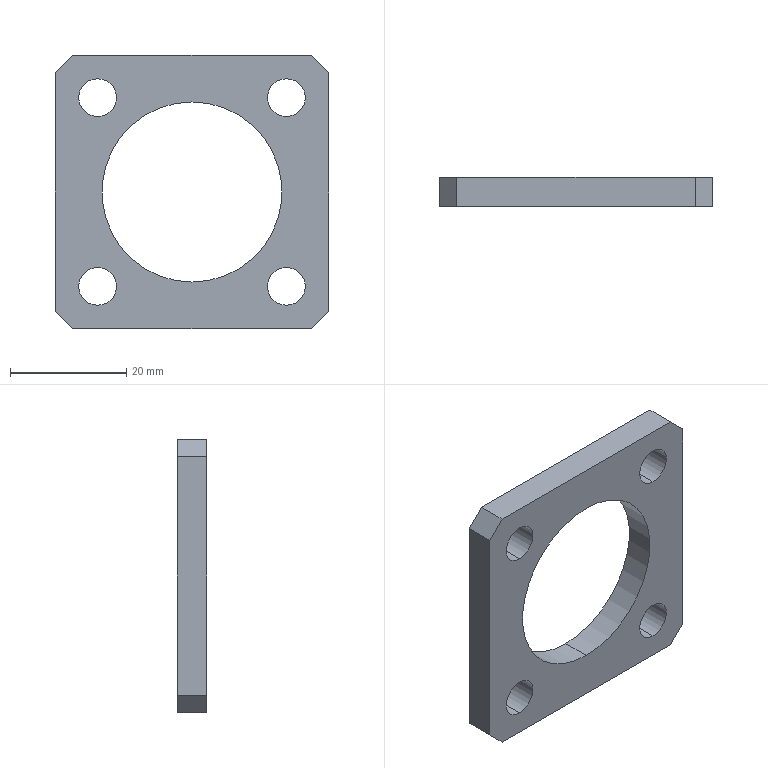Component | SolidWorks | F12529-M5116-1 | 1 solid | 20 faces | box 47 x 5 x 47 mm | volume 6518 mm3 | cylinder 10 | plane 10 | commonest cylinder face diameters 6.5 x8 31 x2
build123d program:
from build123d import *

# Parameters (mm, degrees)
SKETCH1_W           = 47
SKETCH1_H           = 47
BOSS_EXTRUDE1_DEPTH = 5
CHAMFER1_SIZE       = 3
SKETCH2_R           = 15.5
CUT_EXTRUDE1_DEPTH  = 5
SKETCH3_R           = 3.25
CUT_EXTRUDE2_DEPTH  = 5


with BuildPart() as part:
    # Sketch1 → Boss-Extrude1 (new body)
    with BuildSketch(Plane(origin=(0, 0, 0), x_dir=(1, 0, 0), z_dir=(0, 1, 0))):
        Rectangle(SKETCH1_W, SKETCH1_H)
    extrude(amount=BOSS_EXTRUDE1_DEPTH)

    # Chamfer1
    chamfer1_edges = [part.edges().sort_by_distance(p)[0] for p in [
        (-23.5, 2.5, -23.5),
        (23.5, 2.5, -23.5),
        (23.5, 2.5, 23.5),
        (-23.5, 2.5, 23.5),
    ]]
    chamfer(chamfer1_edges, length=CHAMFER1_SIZE)

    # Sketch2 → Cut-Extrude1 (cut)
    with BuildSketch(Plane(origin=(0, 5, 0), x_dir=(1, 0, 0), z_dir=(0, 1, 0))):
        with Locations(Location((0, 0, 0), (0, 0, 270))):
            Circle(SKETCH2_R)
    extrude(amount=-CUT_EXTRUDE1_DEPTH, mode=Mode.SUBTRACT)

    # Sketch3 → Cut-Extrude2 (cut)
    with BuildSketch(Plane(origin=(0, 5, 0), x_dir=(1, 0, 0), z_dir=(0, 1, 0))):
        with Locations(Location((16.25, 16.25, 0), (0, 0, 270))):
            Circle(SKETCH3_R)
        with Locations(Location((16.25, -16.25, 0), (0, 0, 270))):
            Circle(SKETCH3_R)
    cut_extrude2 = extrude(amount=-CUT_EXTRUDE2_DEPTH, mode=Mode.SUBTRACT)

    # Mirror1: Cut-Extrude2 across plane
    add(cut_extrude2.mirror(Plane(origin=(0, 0, 0), x_dir=(0, 0, 1), z_dir=(1, 0, 0))), mode=Mode.SUBTRACT)


solid = part.part

# Placed as in the assembly
solid = solid.moved(Location((0, -5, 0), (0, 0, 0)))
STEP:
#1=COLOUR_RGB('',0.7922,0.8196,0.9333);
#2=FILL_AREA_STYLE_COLOUR('',#1);
#3=FILL_AREA_STYLE('',(#2));
#4=SURFACE_STYLE_FILL_AREA(#3);
#5=SURFACE_SIDE_STYLE('',(#4));
#6=SURFACE_STYLE_USAGE(.BOTH.,#5);
#7=PRESENTATION_STYLE_ASSIGNMENT((#6));
#8=CARTESIAN_POINT('',(-0.6398,-0.1969,0.7677));
#9=VERTEX_POINT('',#8);
#10=CARTESIAN_POINT('',(-0.6398,-0.1969,0.5118));
#11=VERTEX_POINT('',#10);
#12=CARTESIAN_POINT('',(-0.6398,-0.1969,0.6398));
#13=DIRECTION('',(0.,-1.,0.));
#14=DIRECTION('',(0.,0.,1.));
#15=AXIS2_PLACEMENT_3D('',#12,#13,#14);
#16=CIRCLE('',#15,0.128);
#17=EDGE_CURVE('',#9,#11,#16,.T.);
#18=ORIENTED_EDGE('',*,*,#17,.T.);
#19=CARTESIAN_POINT('',(-0.6398,0.,0.5118));
#20=VERTEX_POINT('',#19);
#21=CARTESIAN_POINT('',(-0.6398,-0.1969,0.5118));
#22=DIRECTION('',(0.,1.,0.));
#23=VECTOR('',#22,39.37);
#24=LINE('',#21,#23);
#25=EDGE_CURVE('',#11,#20,#24,.T.);
#26=ORIENTED_EDGE('',*,*,#25,.T.);
#27=CARTESIAN_POINT('',(-0.6398,0.,0.7677));
#28=VERTEX_POINT('',#27);
#29=CARTESIAN_POINT('',(-0.6398,0.,0.6398));
#30=DIRECTION('',(0.,-1.,0.));
#31=DIRECTION('',(0.,0.,1.));
#32=AXIS2_PLACEMENT_3D('',#29,#30,#31);
#33=CIRCLE('',#32,0.128);
#34=EDGE_CURVE('',#28,#20,#33,.T.);
#35=ORIENTED_EDGE('',*,*,#34,.F.);
#36=CARTESIAN_POINT('',(-0.6398,-0.1969,0.7677));
#37=DIRECTION('',(0.,1.,0.));
#38=VECTOR('',#37,39.37);
#39=LINE('',#36,#38);
#40=EDGE_CURVE('',#9,#28,#39,.T.);
#41=ORIENTED_EDGE('',*,*,#40,.F.);
#42=EDGE_LOOP('',(#18,#26,#35,#41));
#43=FACE_OUTER_BOUND('',#42,.T.);
#44=CARTESIAN_POINT('',(-0.6398,-0.1969,0.6398));
#45=DIRECTION('',(0.,1.,0.));
#46=DIRECTION('',(0.,0.,1.));
#47=AXIS2_PLACEMENT_3D('',#44,#45,#46);
#48=CYLINDRICAL_SURFACE('',#47,0.128);
#49=ADVANCED_FACE('',(#43),#48,.F.);
#50=CARTESIAN_POINT('',(-0.6398,-0.1969,-0.5118));
#51=VERTEX_POINT('',#50);
#52=CARTESIAN_POINT('',(-0.6398,-0.1969,-0.7677));
#53=VERTEX_POINT('',#52);
#54=CARTESIAN_POINT('',(-0.6398,-0.1969,-0.6398));
#55=DIRECTION('',(0.,-1.,0.));
#56=DIRECTION('',(0.,0.,1.));
#57=AXIS2_PLACEMENT_3D('',#54,#55,#56);
#58=CIRCLE('',#57,0.128);
#59=EDGE_CURVE('',#51,#53,#58,.T.);
#60=ORIENTED_EDGE('',*,*,#59,.T.);
#61=CARTESIAN_POINT('',(-0.6398,0.,-0.7677));
#62=VERTEX_POINT('',#61);
#63=CARTESIAN_POINT('',(-0.6398,-0.1969,-0.7677));
#64=DIRECTION('',(0.,1.,0.));
#65=VECTOR('',#64,39.37);
#66=LINE('',#63,#65);
#67=EDGE_CURVE('',#53,#62,#66,.T.);
#68=ORIENTED_EDGE('',*,*,#67,.T.);
#69=CARTESIAN_POINT('',(-0.6398,0.,-0.5118));
#70=VERTEX_POINT('',#69);
#71=CARTESIAN_POINT('',(-0.6398,0.,-0.6398));
#72=DIRECTION('',(0.,-1.,0.));
#73=DIRECTION('',(0.,0.,1.));
#74=AXIS2_PLACEMENT_3D('',#71,#72,#73);
#75=CIRCLE('',#74,0.128);
#76=EDGE_CURVE('',#70,#62,#75,.T.);
#77=ORIENTED_EDGE('',*,*,#76,.F.);
#78=CARTESIAN_POINT('',(-0.6398,-0.1969,-0.5118));
#79=DIRECTION('',(0.,1.,0.));
#80=VECTOR('',#79,39.37);
#81=LINE('',#78,#80);
#82=EDGE_CURVE('',#51,#70,#81,.T.);
#83=ORIENTED_EDGE('',*,*,#82,.F.);
#84=EDGE_LOOP('',(#60,#68,#77,#83));
#85=FACE_OUTER_BOUND('',#84,.T.);
#86=CARTESIAN_POINT('',(-0.6398,-0.1969,-0.6398));
#87=DIRECTION('',(0.,1.,0.));
#88=DIRECTION('',(0.,0.,1.));
#89=AXIS2_PLACEMENT_3D('',#86,#87,#88);
#90=CYLINDRICAL_SURFACE('',#89,0.128);
#91=ADVANCED_FACE('',(#85),#90,.F.);
#92=CARTESIAN_POINT('',(0.6398,-0.1969,0.5118));
#93=VERTEX_POINT('',#92);
#94=CARTESIAN_POINT('',(0.6398,-0.1969,0.7677));
#95=VERTEX_POINT('',#94);
#96=CARTESIAN_POINT('',(0.6398,-0.1969,0.6398));
#97=DIRECTION('',(0.,1.,0.));
#98=DIRECTION('',(0.,0.,1.));
#99=AXIS2_PLACEMENT_3D('',#96,#97,#98);
#100=CIRCLE('',#99,0.128);
#101=EDGE_CURVE('',#93,#95,#100,.T.);
#102=ORIENTED_EDGE('',*,*,#101,.F.);
#103=CARTESIAN_POINT('',(0.6398,0.,0.5118));
#104=VERTEX_POINT('',#103);
#105=CARTESIAN_POINT('',(0.6398,-0.1969,0.5118));
#106=DIRECTION('',(0.,1.,0.));
#107=VECTOR('',#106,39.37);
#108=LINE('',#105,#107);
#109=EDGE_CURVE('',#93,#104,#108,.T.);
#110=ORIENTED_EDGE('',*,*,#109,.T.);
#111=CARTESIAN_POINT('',(0.6398,0.,0.7677));
#112=VERTEX_POINT('',#111);
#113=CARTESIAN_POINT('',(0.6398,0.,0.6398));
#114=DIRECTION('',(0.,1.,0.));
#115=DIRECTION('',(0.,0.,1.));
#116=AXIS2_PLACEMENT_3D('',#113,#114,#115);
#117=CIRCLE('',#116,0.128);
#118=EDGE_CURVE('',#104,#112,#117,.T.);
#119=ORIENTED_EDGE('',*,*,#118,.T.);
#120=CARTESIAN_POINT('',(0.6398,-0.1969,0.7677));
#121=DIRECTION('',(0.,1.,0.));
#122=VECTOR('',#121,39.37);
#123=LINE('',#120,#122);
#124=EDGE_CURVE('',#95,#112,#123,.T.);
#125=ORIENTED_EDGE('',*,*,#124,.F.);
#126=EDGE_LOOP('',(#102,#110,#119,#125));
#127=FACE_OUTER_BOUND('',#126,.T.);
#128=CARTESIAN_POINT('',(0.6398,-0.1969,0.6398));
#129=DIRECTION('',(0.,1.,0.));
#130=DIRECTION('',(0.,0.,1.));
#131=AXIS2_PLACEMENT_3D('',#128,#129,#130);
#132=CYLINDRICAL_SURFACE('',#131,0.128);
#133=ADVANCED_FACE('',(#127),#132,.F.);
#134=CARTESIAN_POINT('',(0.6398,-0.1969,-0.7677));
#135=VERTEX_POINT('',#134);
#136=CARTESIAN_POINT('',(0.6398,-0.1969,-0.5118));
#137=VERTEX_POINT('',#136);
#138=CARTESIAN_POINT('',(0.6398,-0.1969,-0.6398));
#139=DIRECTION('',(0.,1.,0.));
#140=DIRECTION('',(0.,0.,1.));
#141=AXIS2_PLACEMENT_3D('',#138,#139,#140);
#142=CIRCLE('',#141,0.128);
#143=EDGE_CURVE('',#135,#137,#142,.T.);
#144=ORIENTED_EDGE('',*,*,#143,.F.);
#145=CARTESIAN_POINT('',(0.6398,0.,-0.7677));
#146=VERTEX_POINT('',#145);
#147=CARTESIAN_POINT('',(0.6398,-0.1969,-0.7677));
#148=DIRECTION('',(0.,1.,0.));
#149=VECTOR('',#148,39.37);
#150=LINE('',#147,#149);
#151=EDGE_CURVE('',#135,#146,#150,.T.);
#152=ORIENTED_EDGE('',*,*,#151,.T.);
#153=CARTESIAN_POINT('',(0.6398,0.,-0.5118));
#154=VERTEX_POINT('',#153);
#155=CARTESIAN_POINT('',(0.6398,0.,-0.6398));
#156=DIRECTION('',(0.,1.,0.));
#157=DIRECTION('',(0.,0.,1.));
#158=AXIS2_PLACEMENT_3D('',#155,#156,#157);
#159=CIRCLE('',#158,0.128);
#160=EDGE_CURVE('',#146,#154,#159,.T.);
#161=ORIENTED_EDGE('',*,*,#160,.T.);
#162=CARTESIAN_POINT('',(0.6398,-0.1969,-0.5118));
#163=DIRECTION('',(0.,1.,0.));
#164=VECTOR('',#163,39.37);
#165=LINE('',#162,#164);
#166=EDGE_CURVE('',#137,#154,#165,.T.);
#167=ORIENTED_EDGE('',*,*,#166,.F.);
#168=EDGE_LOOP('',(#144,#152,#161,#167));
#169=FACE_OUTER_BOUND('',#168,.T.);
#170=CARTESIAN_POINT('',(0.6398,-0.1969,-0.6398));
#171=DIRECTION('',(0.,1.,0.));
#172=DIRECTION('',(0.,0.,1.));
#173=AXIS2_PLACEMENT_3D('',#170,#171,#172);
#174=CYLINDRICAL_SURFACE('',#173,0.128);
#175=ADVANCED_FACE('',(#169),#174,.F.);
#176=CARTESIAN_POINT('',(0.,-0.1969,-0.6102));
#177=VERTEX_POINT('',#176);
#178=CARTESIAN_POINT('',(-0.,-0.1969,0.6102));
#179=VERTEX_POINT('',#178);
#180=CARTESIAN_POINT('',(-0.,-0.1969,-0.));
#181=DIRECTION('',(0.,1.,0.));
#182=DIRECTION('',(0.,0.,1.));
#183=AXIS2_PLACEMENT_3D('',#180,#181,#182);
#184=CIRCLE('',#183,0.6102);
#185=EDGE_CURVE('',#177,#179,#184,.T.);
#186=ORIENTED_EDGE('',*,*,#185,.F.);
#187=CARTESIAN_POINT('',(0.,0.,-0.6102));
#188=VERTEX_POINT('',#187);
#189=CARTESIAN_POINT('',(0.,-0.1969,-0.6102));
#190=DIRECTION('',(0.,1.,0.));
#191=VECTOR('',#190,39.37);
#192=LINE('',#189,#191);
#193=EDGE_CURVE('',#177,#188,#192,.T.);
#194=ORIENTED_EDGE('',*,*,#193,.T.);
#195=CARTESIAN_POINT('',(-0.,0.,0.6102));
#196=VERTEX_POINT('',#195);
#197=CARTESIAN_POINT('',(-0.,0.,-0.));
#198=DIRECTION('',(0.,1.,0.));
#199=DIRECTION('',(0.,0.,1.));
#200=AXIS2_PLACEMENT_3D('',#197,#198,#199);
#201=CIRCLE('',#200,0.6102);
#202=EDGE_CURVE('',#188,#196,#201,.T.);
#203=ORIENTED_EDGE('',*,*,#202,.T.);
#204=CARTESIAN_POINT('',(-0.,-0.1969,0.6102));
#205=DIRECTION('',(0.,1.,0.));
#206=VECTOR('',#205,39.37);
#207=LINE('',#204,#206);
#208=EDGE_CURVE('',#179,#196,#207,.T.);
#209=ORIENTED_EDGE('',*,*,#208,.F.);
#210=EDGE_LOOP('',(#186,#194,#203,#209));
#211=FACE_OUTER_BOUND('',#210,.T.);
#212=CARTESIAN_POINT('',(-0.,-0.1969,-0.));
#213=DIRECTION('',(0.,1.,0.));
#214=DIRECTION('',(0.,0.,1.));
#215=AXIS2_PLACEMENT_3D('',#212,#213,#214);
#216=CYLINDRICAL_SURFACE('',#215,0.6102);
#217=ADVANCED_FACE('',(#211),#216,.F.);
#218=ORIENTED_EDGE('',*,*,#76,.T.);
#219=CARTESIAN_POINT('',(-0.6398,0.,-0.6398));
#220=DIRECTION('',(0.,-1.,0.));
#221=DIRECTION('',(0.,0.,1.));
#222=AXIS2_PLACEMENT_3D('',#219,#220,#221);
#223=CIRCLE('',#222,0.128);
#224=EDGE_CURVE('',#62,#70,#223,.T.);
#225=ORIENTED_EDGE('',*,*,#224,.T.);
#226=EDGE_LOOP('',(#218,#225));
#227=FACE_BOUND('',#226,.T.);
#228=CARTESIAN_POINT('',(0.6398,0.,0.6398));
#229=DIRECTION('',(0.,1.,0.));
#230=DIRECTION('',(0.,0.,1.));
#231=AXIS2_PLACEMENT_3D('',#228,#229,#230);
#232=CIRCLE('',#231,0.128);
#233=EDGE_CURVE('',#112,#104,#232,.T.);
#234=ORIENTED_EDGE('',*,*,#233,.F.);
#235=ORIENTED_EDGE('',*,*,#118,.F.);
#236=EDGE_LOOP('',(#234,#235));
#237=FACE_BOUND('',#236,.T.);
#238=CARTESIAN_POINT('',(0.6398,0.,-0.6398));
#239=DIRECTION('',(0.,1.,0.));
#240=DIRECTION('',(0.,0.,1.));
#241=AXIS2_PLACEMENT_3D('',#238,#239,#240);
#242=CIRCLE('',#241,0.128);
#243=EDGE_CURVE('',#154,#146,#242,.T.);
#244=ORIENTED_EDGE('',*,*,#243,.F.);
#245=ORIENTED_EDGE('',*,*,#160,.F.);
#246=EDGE_LOOP('',(#244,#245));
#247=FACE_BOUND('',#246,.T.);
#248=CARTESIAN_POINT('',(-0.,0.,-0.));
#249=DIRECTION('',(0.,1.,0.));
#250=DIRECTION('',(0.,0.,1.));
#251=AXIS2_PLACEMENT_3D('',#248,#249,#250);
#252=CIRCLE('',#251,0.6102);
#253=EDGE_CURVE('',#196,#188,#252,.T.);
#254=ORIENTED_EDGE('',*,*,#253,.F.);
#255=ORIENTED_EDGE('',*,*,#202,.F.);
#256=EDGE_LOOP('',(#254,#255));
#257=FACE_BOUND('',#256,.T.);
#258=CARTESIAN_POINT('',(-0.9252,0.,-0.8071));
#259=VERTEX_POINT('',#258);
#260=CARTESIAN_POINT('',(-0.9252,0.,0.8071));
#261=VERTEX_POINT('',#260);
#262=CARTESIAN_POINT('',(-0.9252,0.,-0.9252));
#263=DIRECTION('',(0.,0.,1.));
#264=VECTOR('',#263,39.37);
#265=LINE('',#262,#264);
#266=EDGE_CURVE('',#259,#261,#265,.T.);
#267=ORIENTED_EDGE('',*,*,#266,.T.);
#268=CARTESIAN_POINT('',(-0.8071,0.,0.9252));
#269=VERTEX_POINT('',#268);
#270=CARTESIAN_POINT('',(-0.8661,0.,0.8661));
#271=DIRECTION('',(0.7071,0.,0.7071));
#272=VECTOR('',#271,39.37);
#273=LINE('',#270,#272);
#274=EDGE_CURVE('',#261,#269,#273,.T.);
#275=ORIENTED_EDGE('',*,*,#274,.T.);
#276=CARTESIAN_POINT('',(0.8071,0.,0.9252));
#277=VERTEX_POINT('',#276);
#278=CARTESIAN_POINT('',(-0.9252,0.,0.9252));
#279=DIRECTION('',(1.,0.,0.));
#280=VECTOR('',#279,39.37);
#281=LINE('',#278,#280);
#282=EDGE_CURVE('',#269,#277,#281,.T.);
#283=ORIENTED_EDGE('',*,*,#282,.T.);
#284=CARTESIAN_POINT('',(0.9252,0.,0.8071));
#285=VERTEX_POINT('',#284);
#286=CARTESIAN_POINT('',(-0.05906,0.,1.791));
#287=DIRECTION('',(0.7071,0.,-0.7071));
#288=VECTOR('',#287,39.37);
#289=LINE('',#286,#288);
#290=EDGE_CURVE('',#277,#285,#289,.T.);
#291=ORIENTED_EDGE('',*,*,#290,.T.);
#292=CARTESIAN_POINT('',(0.9252,0.,-0.8071));
#293=VERTEX_POINT('',#292);
#294=CARTESIAN_POINT('',(0.9252,0.,-0.9252));
#295=DIRECTION('',(-0.,0.,-1.));
#296=VECTOR('',#295,39.37);
#297=LINE('',#294,#296);
#298=EDGE_CURVE('',#285,#293,#297,.T.);
#299=ORIENTED_EDGE('',*,*,#298,.T.);
#300=CARTESIAN_POINT('',(0.8071,0.,-0.9252));
#301=VERTEX_POINT('',#300);
#302=CARTESIAN_POINT('',(0.8661,0.,-0.8661));
#303=DIRECTION('',(-0.7071,0.,-0.7071));
#304=VECTOR('',#303,39.37);
#305=LINE('',#302,#304);
#306=EDGE_CURVE('',#293,#301,#305,.T.);
#307=ORIENTED_EDGE('',*,*,#306,.T.);
#308=CARTESIAN_POINT('',(-0.8071,0.,-0.9252));
#309=VERTEX_POINT('',#308);
#310=CARTESIAN_POINT('',(-0.9252,0.,-0.9252));
#311=DIRECTION('',(-1.,0.,0.));
#312=VECTOR('',#311,39.37);
#313=LINE('',#310,#312);
#314=EDGE_CURVE('',#301,#309,#313,.T.);
#315=ORIENTED_EDGE('',*,*,#314,.T.);
#316=CARTESIAN_POINT('',(-1.791,0.,0.05906));
#317=DIRECTION('',(-0.7071,0.,0.7071));
#318=VECTOR('',#317,39.37);
#319=LINE('',#316,#318);
#320=EDGE_CURVE('',#309,#259,#319,.T.);
#321=ORIENTED_EDGE('',*,*,#320,.T.);
#322=EDGE_LOOP('',(#267,#275,#283,#291,#299,#307,#315,#321));
#323=FACE_OUTER_BOUND('',#322,.T.);
#324=ORIENTED_EDGE('',*,*,#34,.T.);
#325=CARTESIAN_POINT('',(-0.6398,0.,0.6398));
#326=DIRECTION('',(0.,-1.,0.));
#327=DIRECTION('',(0.,0.,1.));
#328=AXIS2_PLACEMENT_3D('',#325,#326,#327);
#329=CIRCLE('',#328,0.128);
#330=EDGE_CURVE('',#20,#28,#329,.T.);
#331=ORIENTED_EDGE('',*,*,#330,.T.);
#332=EDGE_LOOP('',(#324,#331));
#333=FACE_BOUND('',#332,.T.);
#334=CARTESIAN_POINT('',(-0.9252,0.,0.9252));
#335=DIRECTION('',(0.,1.,0.));
#336=DIRECTION('',(0.,0.,1.));
#337=AXIS2_PLACEMENT_3D('',#334,#335,#336);
#338=PLANE('',#337);
#339=ADVANCED_FACE('',(#227,#237,#247,#257,#323,#333),#338,.T.);
#340=CARTESIAN_POINT('',(0.6398,-0.1969,0.6398));
#341=DIRECTION('',(0.,1.,0.));
#342=DIRECTION('',(0.,0.,1.));
#343=AXIS2_PLACEMENT_3D('',#340,#341,#342);
#344=CIRCLE('',#343,0.128);
#345=EDGE_CURVE('',#95,#93,#344,.T.);
#346=ORIENTED_EDGE('',*,*,#345,.T.);
#347=ORIENTED_EDGE('',*,*,#101,.T.);
#348=EDGE_LOOP('',(#346,#347));
#349=FACE_BOUND('',#348,.T.);
#350=CARTESIAN_POINT('',(0.6398,-0.1969,-0.6398));
#351=DIRECTION('',(0.,1.,0.));
#352=DIRECTION('',(0.,0.,1.));
#353=AXIS2_PLACEMENT_3D('',#350,#351,#352);
#354=CIRCLE('',#353,0.128);
#355=EDGE_CURVE('',#137,#135,#354,.T.);
#356=ORIENTED_EDGE('',*,*,#355,.T.);
#357=ORIENTED_EDGE('',*,*,#143,.T.);
#358=EDGE_LOOP('',(#356,#357));
#359=FACE_BOUND('',#358,.T.);
#360=CARTESIAN_POINT('',(-0.,-0.1969,-0.));
#361=DIRECTION('',(0.,1.,0.));
#362=DIRECTION('',(0.,0.,1.));
#363=AXIS2_PLACEMENT_3D('',#360,#361,#362);
#364=CIRCLE('',#363,0.6102);
#365=EDGE_CURVE('',#179,#177,#364,.T.);
#366=ORIENTED_EDGE('',*,*,#365,.T.);
#367=ORIENTED_EDGE('',*,*,#185,.T.);
#368=EDGE_LOOP('',(#366,#367));
#369=FACE_BOUND('',#368,.T.);
#370=CARTESIAN_POINT('',(-0.8071,-0.1969,0.9252));
#371=VERTEX_POINT('',#370);
#372=CARTESIAN_POINT('',(0.8071,-0.1969,0.9252));
#373=VERTEX_POINT('',#372);
#374=CARTESIAN_POINT('',(-0.9252,-0.1969,0.9252));
#375=DIRECTION('',(1.,0.,0.));
#376=VECTOR('',#375,39.37);
#377=LINE('',#374,#376);
#378=EDGE_CURVE('',#371,#373,#377,.T.);
#379=ORIENTED_EDGE('',*,*,#378,.F.);
#380=CARTESIAN_POINT('',(-0.9252,-0.1969,0.8071));
#381=VERTEX_POINT('',#380);
#382=CARTESIAN_POINT('',(-0.8071,-0.1969,0.9252));
#383=DIRECTION('',(-0.7071,0.,-0.7071));
#384=VECTOR('',#383,39.37);
#385=LINE('',#382,#384);
#386=EDGE_CURVE('',#371,#381,#385,.T.);
#387=ORIENTED_EDGE('',*,*,#386,.T.);
#388=CARTESIAN_POINT('',(-0.9252,-0.1969,-0.8071));
#389=VERTEX_POINT('',#388);
#390=CARTESIAN_POINT('',(-0.9252,-0.1969,-0.9252));
#391=DIRECTION('',(0.,0.,1.));
#392=VECTOR('',#391,39.37);
#393=LINE('',#390,#392);
#394=EDGE_CURVE('',#389,#381,#393,.T.);
#395=ORIENTED_EDGE('',*,*,#394,.F.);
#396=CARTESIAN_POINT('',(-0.8071,-0.1969,-0.9252));
#397=VERTEX_POINT('',#396);
#398=CARTESIAN_POINT('',(-0.9252,-0.1969,-0.8071));
#399=DIRECTION('',(0.7071,0.,-0.7071));
#400=VECTOR('',#399,39.37);
#401=LINE('',#398,#400);
#402=EDGE_CURVE('',#389,#397,#401,.T.);
#403=ORIENTED_EDGE('',*,*,#402,.T.);
#404=CARTESIAN_POINT('',(0.8071,-0.1969,-0.9252));
#405=VERTEX_POINT('',#404);
#406=CARTESIAN_POINT('',(-0.9252,-0.1969,-0.9252));
#407=DIRECTION('',(-1.,0.,0.));
#408=VECTOR('',#407,39.37);
#409=LINE('',#406,#408);
#410=EDGE_CURVE('',#405,#397,#409,.T.);
#411=ORIENTED_EDGE('',*,*,#410,.F.);
#412=CARTESIAN_POINT('',(0.9252,-0.1969,-0.8071));
#413=VERTEX_POINT('',#412);
#414=CARTESIAN_POINT('',(0.8071,-0.1969,-0.9252));
#415=DIRECTION('',(0.7071,0.,0.7071));
#416=VECTOR('',#415,39.37);
#417=LINE('',#414,#416);
#418=EDGE_CURVE('',#405,#413,#417,.T.);
#419=ORIENTED_EDGE('',*,*,#418,.T.);
#420=CARTESIAN_POINT('',(0.9252,-0.1969,0.8071));
#421=VERTEX_POINT('',#420);
#422=CARTESIAN_POINT('',(0.9252,-0.1969,-0.9252));
#423=DIRECTION('',(-0.,0.,-1.));
#424=VECTOR('',#423,39.37);
#425=LINE('',#422,#424);
#426=EDGE_CURVE('',#421,#413,#425,.T.);
#427=ORIENTED_EDGE('',*,*,#426,.F.);
#428=CARTESIAN_POINT('',(0.9252,-0.1969,0.8071));
#429=DIRECTION('',(-0.7071,0.,0.7071));
#430=VECTOR('',#429,39.37);
#431=LINE('',#428,#430);
#432=EDGE_CURVE('',#421,#373,#431,.T.);
#433=ORIENTED_EDGE('',*,*,#432,.T.);
#434=EDGE_LOOP('',(#379,#387,#395,#403,#411,#419,#427,#433));
#435=FACE_OUTER_BOUND('',#434,.T.);
#436=ORIENTED_EDGE('',*,*,#59,.F.);
#437=CARTESIAN_POINT('',(-0.6398,-0.1969,-0.6398));
#438=DIRECTION('',(0.,-1.,0.));
#439=DIRECTION('',(0.,0.,1.));
#440=AXIS2_PLACEMENT_3D('',#437,#438,#439);
#441=CIRCLE('',#440,0.128);
#442=EDGE_CURVE('',#53,#51,#441,.T.);
#443=ORIENTED_EDGE('',*,*,#442,.F.);
#444=EDGE_LOOP('',(#436,#443));
#445=FACE_BOUND('',#444,.T.);
#446=ORIENTED_EDGE('',*,*,#17,.F.);
#447=CARTESIAN_POINT('',(-0.6398,-0.1969,0.6398));
#448=DIRECTION('',(0.,-1.,0.));
#449=DIRECTION('',(0.,0.,1.));
#450=AXIS2_PLACEMENT_3D('',#447,#448,#449);
#451=CIRCLE('',#450,0.128);
#452=EDGE_CURVE('',#11,#9,#451,.T.);
#453=ORIENTED_EDGE('',*,*,#452,.F.);
#454=EDGE_LOOP('',(#446,#453));
#455=FACE_BOUND('',#454,.T.);
#456=CARTESIAN_POINT('',(-0.9252,-0.1969,0.9252));
#457=DIRECTION('',(0.,1.,0.));
#458=DIRECTION('',(0.,0.,1.));
#459=AXIS2_PLACEMENT_3D('',#456,#457,#458);
#460=PLANE('',#459);
#461=ADVANCED_FACE('',(#349,#359,#369,#435,#445,#455),#460,.F.);
#462=ORIENTED_EDGE('',*,*,#394,.T.);
#463=CARTESIAN_POINT('',(-0.9252,0.,0.8071));
#464=DIRECTION('',(0.,1.,0.));
#465=VECTOR('',#464,39.37);
#466=LINE('',#463,#465);
#467=EDGE_CURVE('',#381,#261,#466,.T.);
#468=ORIENTED_EDGE('',*,*,#467,.T.);
#469=ORIENTED_EDGE('',*,*,#266,.F.);
#470=CARTESIAN_POINT('',(-0.9252,0.,-0.8071));
#471=DIRECTION('',(0.,-1.,0.));
#472=VECTOR('',#471,39.37);
#473=LINE('',#470,#472);
#474=EDGE_CURVE('',#259,#389,#473,.T.);
#475=ORIENTED_EDGE('',*,*,#474,.T.);
#476=EDGE_LOOP('',(#462,#468,#469,#475));
#477=FACE_OUTER_BOUND('',#476,.T.);
#478=CARTESIAN_POINT('',(-0.9252,0.,-0.9252));
#479=DIRECTION('',(1.,0.,-0.));
#480=DIRECTION('',(-0.,0.,-1.));
#481=AXIS2_PLACEMENT_3D('',#478,#479,#480);
#482=PLANE('',#481);
#483=ADVANCED_FACE('',(#477),#482,.F.);
#484=ORIENTED_EDGE('',*,*,#282,.F.);
#485=CARTESIAN_POINT('',(-0.8071,0.,0.9252));
#486=DIRECTION('',(0.,-1.,0.));
#487=VECTOR('',#486,39.37);
#488=LINE('',#485,#487);
#489=EDGE_CURVE('',#269,#371,#488,.T.);
#490=ORIENTED_EDGE('',*,*,#489,.T.);
#491=ORIENTED_EDGE('',*,*,#378,.T.);
#492=CARTESIAN_POINT('',(0.8071,0.,0.9252));
#493=DIRECTION('',(0.,1.,0.));
#494=VECTOR('',#493,39.37);
#495=LINE('',#492,#494);
#496=EDGE_CURVE('',#373,#277,#495,.T.);
#497=ORIENTED_EDGE('',*,*,#496,.T.);
#498=EDGE_LOOP('',(#484,#490,#491,#497));
#499=FACE_OUTER_BOUND('',#498,.T.);
#500=CARTESIAN_POINT('',(-0.9252,0.,0.9252));
#501=DIRECTION('',(0.,0.,-1.));
#502=DIRECTION('',(-1.,0.,0.));
#503=AXIS2_PLACEMENT_3D('',#500,#501,#502);
#504=PLANE('',#503);
#505=ADVANCED_FACE('',(#499),#504,.F.);
#506=ORIENTED_EDGE('',*,*,#426,.T.);
#507=CARTESIAN_POINT('',(0.9252,0.,-0.8071));
#508=DIRECTION('',(0.,1.,0.));
#509=VECTOR('',#508,39.37);
#510=LINE('',#507,#509);
#511=EDGE_CURVE('',#413,#293,#510,.T.);
#512=ORIENTED_EDGE('',*,*,#511,.T.);
#513=ORIENTED_EDGE('',*,*,#298,.F.);
#514=CARTESIAN_POINT('',(0.9252,0.,0.8071));
#515=DIRECTION('',(0.,-1.,0.));
#516=VECTOR('',#515,39.37);
#517=LINE('',#514,#516);
#518=EDGE_CURVE('',#285,#421,#517,.T.);
#519=ORIENTED_EDGE('',*,*,#518,.T.);
#520=EDGE_LOOP('',(#506,#512,#513,#519));
#521=FACE_OUTER_BOUND('',#520,.T.);
#522=CARTESIAN_POINT('',(0.9252,0.,-0.9252));
#523=DIRECTION('',(-1.,0.,0.));
#524=DIRECTION('',(0.,0.,1.));
#525=AXIS2_PLACEMENT_3D('',#522,#523,#524);
#526=PLANE('',#525);
#527=ADVANCED_FACE('',(#521),#526,.F.);
#528=ORIENTED_EDGE('',*,*,#410,.T.);
#529=CARTESIAN_POINT('',(-0.8071,0.,-0.9252));
#530=DIRECTION('',(0.,1.,0.));
#531=VECTOR('',#530,39.37);
#532=LINE('',#529,#531);
#533=EDGE_CURVE('',#397,#309,#532,.T.);
#534=ORIENTED_EDGE('',*,*,#533,.T.);
#535=ORIENTED_EDGE('',*,*,#314,.F.);
#536=CARTESIAN_POINT('',(0.8071,0.,-0.9252));
#537=DIRECTION('',(0.,-1.,0.));
#538=VECTOR('',#537,39.37);
#539=LINE('',#536,#538);
#540=EDGE_CURVE('',#301,#405,#539,.T.);
#541=ORIENTED_EDGE('',*,*,#540,.T.);
#542=EDGE_LOOP('',(#528,#534,#535,#541));
#543=FACE_OUTER_BOUND('',#542,.T.);
#544=CARTESIAN_POINT('',(-0.9252,0.,-0.9252));
#545=DIRECTION('',(0.,0.,1.));
#546=DIRECTION('',(1.,0.,0.));
#547=AXIS2_PLACEMENT_3D('',#544,#545,#546);
#548=PLANE('',#547);
#549=ADVANCED_FACE('',(#543),#548,.F.);
#550=ORIENTED_EDGE('',*,*,#274,.F.);
#551=ORIENTED_EDGE('',*,*,#467,.F.);
#552=ORIENTED_EDGE('',*,*,#386,.F.);
#553=ORIENTED_EDGE('',*,*,#489,.F.);
#554=EDGE_LOOP('',(#550,#551,#552,#553));
#555=FACE_OUTER_BOUND('',#554,.T.);
#556=CARTESIAN_POINT('',(-0.8071,0.,0.9252));
#557=DIRECTION('',(0.7071,0.,-0.7071));
#558=DIRECTION('',(-0.7071,0.,-0.7071));
#559=AXIS2_PLACEMENT_3D('',#556,#557,#558);
#560=PLANE('',#559);
#561=ADVANCED_FACE('',(#555),#560,.F.);
#562=ORIENTED_EDGE('',*,*,#320,.F.);
#563=ORIENTED_EDGE('',*,*,#533,.F.);
#564=ORIENTED_EDGE('',*,*,#402,.F.);
#565=ORIENTED_EDGE('',*,*,#474,.F.);
#566=EDGE_LOOP('',(#562,#563,#564,#565));
#567=FACE_OUTER_BOUND('',#566,.T.);
#568=CARTESIAN_POINT('',(-0.9252,0.,-0.8071));
#569=DIRECTION('',(0.7071,0.,0.7071));
#570=DIRECTION('',(0.7071,0.,-0.7071));
#571=AXIS2_PLACEMENT_3D('',#568,#569,#570);
#572=PLANE('',#571);
#573=ADVANCED_FACE('',(#567),#572,.F.);
#574=ORIENTED_EDGE('',*,*,#306,.F.);
#575=ORIENTED_EDGE('',*,*,#511,.F.);
#576=ORIENTED_EDGE('',*,*,#418,.F.);
#577=ORIENTED_EDGE('',*,*,#540,.F.);
#578=EDGE_LOOP('',(#574,#575,#576,#577));
#579=FACE_OUTER_BOUND('',#578,.T.);
#580=CARTESIAN_POINT('',(0.8071,0.,-0.9252));
#581=DIRECTION('',(-0.7071,0.,0.7071));
#582=DIRECTION('',(0.7071,0.,0.7071));
#583=AXIS2_PLACEMENT_3D('',#580,#581,#582);
#584=PLANE('',#583);
#585=ADVANCED_FACE('',(#579),#584,.F.);
#586=ORIENTED_EDGE('',*,*,#290,.F.);
#587=ORIENTED_EDGE('',*,*,#496,.F.);
#588=ORIENTED_EDGE('',*,*,#432,.F.);
#589=ORIENTED_EDGE('',*,*,#518,.F.);
#590=EDGE_LOOP('',(#586,#587,#588,#589));
#591=FACE_OUTER_BOUND('',#590,.T.);
#592=CARTESIAN_POINT('',(0.9252,0.,0.8071));
#593=DIRECTION('',(-0.7071,0.,-0.7071));
#594=DIRECTION('',(-0.7071,0.,0.7071));
#595=AXIS2_PLACEMENT_3D('',#592,#593,#594);
#596=PLANE('',#595);
#597=ADVANCED_FACE('',(#591),#596,.F.);
#598=ORIENTED_EDGE('',*,*,#193,.F.);
#599=ORIENTED_EDGE('',*,*,#365,.F.);
#600=ORIENTED_EDGE('',*,*,#208,.T.);
#601=ORIENTED_EDGE('',*,*,#253,.T.);
#602=EDGE_LOOP('',(#598,#599,#600,#601));
#603=FACE_OUTER_BOUND('',#602,.T.);
#604=CARTESIAN_POINT('',(-0.,-0.1969,-0.));
#605=DIRECTION('',(0.,1.,0.));
#606=DIRECTION('',(0.,0.,1.));
#607=AXIS2_PLACEMENT_3D('',#604,#605,#606);
#608=CYLINDRICAL_SURFACE('',#607,0.6102);
#609=ADVANCED_FACE('',(#603),#608,.F.);
#610=ORIENTED_EDGE('',*,*,#151,.F.);
#611=ORIENTED_EDGE('',*,*,#355,.F.);
#612=ORIENTED_EDGE('',*,*,#166,.T.);
#613=ORIENTED_EDGE('',*,*,#243,.T.);
#614=EDGE_LOOP('',(#610,#611,#612,#613));
#615=FACE_OUTER_BOUND('',#614,.T.);
#616=CARTESIAN_POINT('',(0.6398,-0.1969,-0.6398));
#617=DIRECTION('',(0.,1.,0.));
#618=DIRECTION('',(0.,0.,1.));
#619=AXIS2_PLACEMENT_3D('',#616,#617,#618);
#620=CYLINDRICAL_SURFACE('',#619,0.128);
#621=ADVANCED_FACE('',(#615),#620,.F.);
#622=ORIENTED_EDGE('',*,*,#109,.F.);
#623=ORIENTED_EDGE('',*,*,#345,.F.);
#624=ORIENTED_EDGE('',*,*,#124,.T.);
#625=ORIENTED_EDGE('',*,*,#233,.T.);
#626=EDGE_LOOP('',(#622,#623,#624,#625));
#627=FACE_OUTER_BOUND('',#626,.T.);
#628=CARTESIAN_POINT('',(0.6398,-0.1969,0.6398));
#629=DIRECTION('',(0.,1.,0.));
#630=DIRECTION('',(0.,0.,1.));
#631=AXIS2_PLACEMENT_3D('',#628,#629,#630);
#632=CYLINDRICAL_SURFACE('',#631,0.128);
#633=ADVANCED_FACE('',(#627),#632,.F.);
#634=ORIENTED_EDGE('',*,*,#67,.F.);
#635=ORIENTED_EDGE('',*,*,#442,.T.);
#636=ORIENTED_EDGE('',*,*,#82,.T.);
#637=ORIENTED_EDGE('',*,*,#224,.F.);
#638=EDGE_LOOP('',(#634,#635,#636,#637));
#639=FACE_OUTER_BOUND('',#638,.T.);
#640=CARTESIAN_POINT('',(-0.6398,-0.1969,-0.6398));
#641=DIRECTION('',(0.,1.,0.));
#642=DIRECTION('',(0.,0.,1.));
#643=AXIS2_PLACEMENT_3D('',#640,#641,#642);
#644=CYLINDRICAL_SURFACE('',#643,0.128);
#645=ADVANCED_FACE('',(#639),#644,.F.);
#646=ORIENTED_EDGE('',*,*,#25,.F.);
#647=ORIENTED_EDGE('',*,*,#452,.T.);
#648=ORIENTED_EDGE('',*,*,#40,.T.);
#649=ORIENTED_EDGE('',*,*,#330,.F.);
#650=EDGE_LOOP('',(#646,#647,#648,#649));
#651=FACE_OUTER_BOUND('',#650,.T.);
#652=CARTESIAN_POINT('',(-0.6398,-0.1969,0.6398));
#653=DIRECTION('',(0.,1.,0.));
#654=DIRECTION('',(0.,0.,1.));
#655=AXIS2_PLACEMENT_3D('',#652,#653,#654);
#656=CYLINDRICAL_SURFACE('',#655,0.128);
#657=ADVANCED_FACE('',(#651),#656,.F.);
#658=CLOSED_SHELL('',(#49,#91,#133,#175,#217,#339,#461,#483,#505,#527,#549,#561,#573,#585,#597,#609,#621,#633,#645,#657));
#659=MANIFOLD_SOLID_BREP('',#658);
#660=STYLED_ITEM('',(#7),#659);
#661=PRESENTATION_LAYER_ASSIGNMENT('','',(#660));
#662=CARTESIAN_POINT('',(0.,0.,0.));
#663=DIRECTION('',(0.,0.,1.));
#664=DIRECTION('',(1.,0.,0.));
#665=AXIS2_PLACEMENT_3D('',#662,#663,#664);
#666=(LENGTH_UNIT()NAMED_UNIT(*)SI_UNIT($,.METRE.));
#667=LENGTH_MEASURE_WITH_UNIT(LENGTH_MEASURE(0.0254),#666);
#668=DIMENSIONAL_EXPONENTS(1.,0.,0.,0.,0.,0.,0.);
#669=(CONVERSION_BASED_UNIT('',#667)LENGTH_UNIT()NAMED_UNIT(#668));
#670=UNCERTAINTY_MEASURE_WITH_UNIT(LENGTH_MEASURE(0.00001),#669,'','');
#671=(NAMED_UNIT(*)PLANE_ANGLE_UNIT()SI_UNIT($,.RADIAN.));
#672=(NAMED_UNIT(*)SI_UNIT($,.STERADIAN.)SOLID_ANGLE_UNIT());
#673=(GEOMETRIC_REPRESENTATION_CONTEXT(3)GLOBAL_UNCERTAINTY_ASSIGNED_CONTEXT((#670))GLOBAL_UNIT_ASSIGNED_CONTEXT((#669,#671,#672))REPRESENTATION_CONTEXT('',''));
#674=ADVANCED_BREP_SHAPE_REPRESENTATION('',(#659,#665),#673);
#675=(LENGTH_UNIT()NAMED_UNIT(*)SI_UNIT($,.METRE.));
#676=LENGTH_MEASURE_WITH_UNIT(LENGTH_MEASURE(0.0254),#675);
#677=DIMENSIONAL_EXPONENTS(1.,0.,0.,0.,0.,0.,0.);
#678=(CONVERSION_BASED_UNIT('',#676)LENGTH_UNIT()NAMED_UNIT(#677));
#679=UNCERTAINTY_MEASURE_WITH_UNIT(LENGTH_MEASURE(0.00001),#678,'','');
#680=(NAMED_UNIT(*)PLANE_ANGLE_UNIT()SI_UNIT($,.RADIAN.));
#681=(NAMED_UNIT(*)SI_UNIT($,.STERADIAN.)SOLID_ANGLE_UNIT());
#682=(GEOMETRIC_REPRESENTATION_CONTEXT(3)GLOBAL_UNCERTAINTY_ASSIGNED_CONTEXT((#679))GLOBAL_UNIT_ASSIGNED_CONTEXT((#678,#680,#681))REPRESENTATION_CONTEXT('',''));
#683=MECHANICAL_DESIGN_GEOMETRIC_PRESENTATION_REPRESENTATION('',(#660),#682);